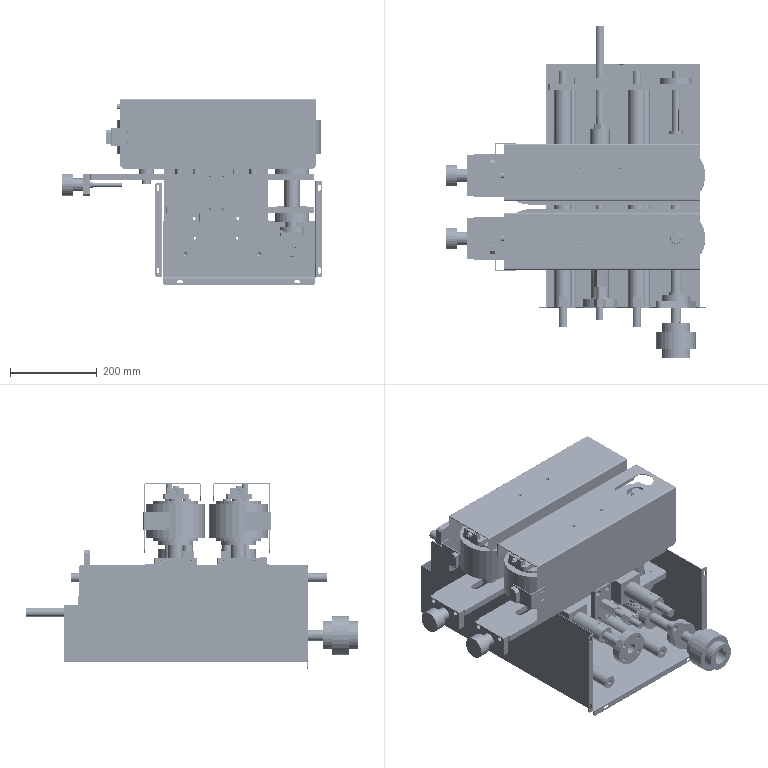Assembly | SolidWorks | mm | 121 component files | 121 solids | 5786 faces | box 600 x 763.5 x 427 mm | volume 18234957 mm3 | cylinder 1615 | torus 1437 | plane 1034 | sphere 814 | spline 504 | cone 382 | commonest cylinder face diameters 11 x120 20 x107 9 x88 17 x76 5 x68 6.8 x66 30 x66 8.5 x64
Bill of materials:
Rolling bearings 6004 GB 276-94 | 13 |  | Annular ring assembly that looks like a radial ball bearing: a thin outer ring and an inner ring, both plain cylinders, sharing an axis, with a single row of spherical balls between them.
'-6004BearingHousing | 1 |  | Flat annular disc with a large central bore and four equally spaced small through holes on a circle between the bore and the outer edge.
ref6 | 8 |  | Ball-bearing-like assembly: concentric outer and inner rings with a single row of about 20 balls between them, and rounded ring edges.
6006BearingHousing | 4 |  | Thick annular ring (spacer- or flange-like shape) with a large central bore and four equally spaced counterbored through holes.
'-BeltTensionBlock | 2 |  | Rectangular block with two counterbored vertical through holes near its ends and one larger horizontal through hole crossing the middle of the long side face.
'-BeltTensionHandwheel | 2 |  | Stepped cylindrical bushing-like part with a larger-diameter section and a coaxial smaller-diameter spigot, with an axial bore visible at the small end.
'-BeltTensionScrewRod | 2 |  | Solid cylindrical pin or shaft with a short, raised, larger-diameter collar near one end. The shaft segments on either side of the collar have slightly different diameters.
'-CoverTopPost | 4 |  | Long slender cylindrical rod with an axial hole at one end and a reduced-diameter stepped spigot at the other end.
'-CylinderConnectionSeat | 1 |  | Block with a T-shaped profile: a wide rectangular top plate with chamfered corners and four vertical through holes, above a narrower lower body that has a horizontal through hole and chamfered lower corners.
deep groove ball bearings gb | 3 |  | Ball-bearing-like assembly: concentric outer and inner rings with a single row of about 14 balls, and rounded ring edges.
'-DrivenPulley | 2 |  | Cylindrical sleeve with a central through bore and a short reduced-outer-diameter step at one end.
'-DrivenPulleyShaft | 2 |  | Multi-stepped shaft with a flatted end tang containing a cross hole, a short collar with a groove-like line, a long main body, a larger-diameter band, and reduced, flatted sections at the opposite end.
'-DrivePulleyStopSleeve | 2 |  | Short, thin-walled cylindrical ring or tube section with plain inner and outer diameters.
'-F-M16150F | 1 |  | Stepped, axially symmetric body: a large chamfered cylinder with a hexagonal prism at one end and a series of smaller coaxial steps leading to a long, slender cylindrical shaft at the other end.
'-GuideBushing | 8 |  | Thin-walled, open-ended cylindrical tube or sleeve of constant diameter.
'-GuidePost | 2 |  | Long, slender cylindrical pin or shaft with reduced-diameter journals at both ends and an extra short shoulder step near one end.
'-LimitScrewRod | 1 |  | Hex-headed rod: a long plain cylindrical shank with a short hexagonal head at one end, in the general form of a hex bolt or screw.
'-LimitScrewSleeve | 1 |  | Flanged tube or spigot: a long cylindrical tube joined to a circular flange with a central bore and four bolt holes.
'-LowerGuard | 1 |  | Bent sheet-metal bracket or cover: a top web with one long side flange and one short side flange (an uneven channel), with small holes and an obround slot.
'-LowerSlideSleeveConnectionPlate01 | 1 |  | Rectangular flat plate with chamfered corners, eight through holes in two 2x2 groups, and a large central hole surrounded by four small holes near one end.
'-LowerSlideSleeveConnectionPlate02 | 1 |  | Long, narrow flat plate with chamfered corners and many features: an elongated slot, several groups of round holes in different sizes, and a large hole with four small holes around it near one end.
'-LowerSlideSleeveConnectionPlate02-1 | 1 |  | Long, narrow flat bar with chamfered corners, an elongated slot and two small holes at one end, two short obround slots and two small round holes along the middle, and a large round hole at the other end.
'-LowerStopBlock | 1 |  | Thick rectangular block or spacer plate with chamfered corners and four through holes near the corners.
M16LocatingScrew | 1 |  | Plain cylindrical rod with a hexagonal collar or nut-like prism at mid-length.
M16Nut | 1 |  | Hexagonal prism with a round through bore along its axis, in the general form of a hex spacer, standoff or coupling sleeve.
'-M30X1.5Nut | 1 |  | Flat, thin annular ring with four rectangular notches cut into the outer edge, spaced evenly around it.
GB_FASTENER_SCREWS_HSHCS M8X60-N | 2 |  | Long, straight cylindrical pin with a short, larger-diameter cylindrical head at one end, like a headed pin or ejector-style pin.
'-MainDrivePulley | 2 |  | Solid cylindrical hub with a central keyed bore and a short, smaller-diameter step at one end.
MaterialDetectionSensor | 2 |  | Rectangular block. Its profile has two rounded corners and one angled corner. Two round holes pass through near one edge.
MaterialDetectionSensorMountingPlate | 2 |  | L-shaped bracket bent from sheet, with a uniform thin wall, an inside bend radius, and two elongated slots in each leg.
'-MovingBushing | 4 |  | Rectangular block with a large round bore running along its long axis and four small holes in a rectangular pattern on one long face.
'-MovingSleeve | 1 |  | Tubular sleeve with a stepped outer diameter, an internal keyway, and a small notch in the outer rim at one end.
ref3 | 3 |  | Straight-tooth bevel gear with a cylindrical hub on its back, a keyed central bore, and small radial holes in the hub.
'-PullerDriveShaft | 1 |  | Long, slender stepped shaft with two main diameters, several keyseats along its length, and chamfered ends.
SC-63X100PistonRod | 1 |  | Stepped cylindrical pin or shaft: a long main body, a short narrow groove or collar near one end, then a smaller-diameter end stub.
'-SlidingBearingHousing | 1 |  | Thick rectangular plate with one large round hole near one end, three small holes in a row at the other end, and two chamfered corners at the large-hole end.
'-SmallPulley | 6 |  | Plain cylindrical tube or sleeve with a uniform outer diameter and a large through-bore.
'-SmallPulleyBearingHousing | 6 |  | Rectangular base plate with two through holes and a centered upright stepped post: a larger-diameter collar, then a long smaller pin with a groove near the tip.
'-SmallSupport | 4 |  | Slender cylindrical rod with a small axial hole in one end face. The other end steps down to a short pin of smaller diameter, and the section next to that pin has a flat cut on one side.
'-SpacerPlate | 1 |  | Rectangular block with three evenly spaced round through-holes in a row across one long side face.
'-TighteningHandwheelBasePlate | 2 |  | Thick rectangular plate with one larger central hole, two smaller holes near the top corners, and chamfered bottom corners.
'-TopPlateSupport | 2 |  | Long thin cylindrical tube or rod with a small concentric hole in the end face.
'-TractionBelt | 2 |  | Thin-walled open loop shaped like a stadium (obround): two straight sides joined by semicircular ends, with a constant wall height and open top and bottom.
ref29 | 1 |  | Straight-tooth bevel gear with a cylindrical hub, a central bore with a keyway, and a small radial hole through the hub.
TractorCoupling | 1 |  | Stepped cylindrical body: a larger-diameter center section with a smaller cylindrical hub on each side, and a central through-bore with a keyway.
'-TractorCover | 1 |  | Sheet-metal tray or enclosure: flat base, two tall side walls with outward mounting flanges that have slotted holes, a lower back wall with a rectangular notch that has rounded corners, and a bottom-edge flange with slots.
'-TractorDriveShaft | 2 |  | Stepped round shaft with several diameter sections: a larger central section, smaller sections stepping down toward one end, and narrow grooves near the other end.
'-TractorTopPlate | 1 |  | Flat L-shaped (stepped) plate with chamfered corners. It has a large central obround slot surrounded by four small holes and four larger corner holes, plus a smaller round hole with four small holes around it on the extended lower portion.
'-UCFL205 | 1 |  | Two-hole diamond-shaped flange with rounded ends, a central through-bore, and a stepped cylindrical boss on one face.
'-UpperGuard | 1 |  | Bent sheet-metal cover with an inverted-U or channel profile: a flat top and two downturned legs of unequal length, with rounded bends.
'-UpperPullCylinderMountingPlate | 1 |  | Rectangular flat plate with small chamfered corners, a large central round through-hole, four round through-holes in a rectangular pattern, and four elongated through-slots (two near each short edge), oriented across the plate's long direction.
'-UpperSlidingSleeveConnectingPlate01 | 1 |  | Elongated rectangular flat plate with small chamfered corners, a large round through-hole near one end surrounded by four small holes in a square pattern, plus several patterns of medium and small through-holes along the rest of the plate.
'-UpperSlidingSleeveConnectingPlate02 | 1 |  | Long narrow flat plate with small chamfered corners. It has one long obround slot near one end, a large round through-hole with four small surrounding holes near the other end, and two roughly mirrored clusters of medium and small round holes in between.
'-UpperSlidingSleeveConnectingPlate02-1 | 1 |  | Long narrow flat bar with chamfered corners. It has a long obround slot near one end with two small holes at that end edge, a central row of two small round holes and two short obround slots, and a large round through-hole near the other end.
Mates:
1. parallel | -GuidePost-3 plane at (-55, 1481, -40) dir (0, 0, 1) | assembly plane at (0, 0, 0) dir (0, 0, 1)
2. parallel | -GuidePost-4 plane at (115, 1481, -40) dir (0, 0, 1) | assembly plane at (0, 0, 0) dir (0, 0, 1)
3. concentric | -GuideBushing-1 face at (-55, 1084.5, -40) dir (0, 1, 0) r 22 | -GuideBushing-2 face at (-55, 1024.5, -40) dir (0, 1, 0) r 22
4. concentric | -MovingBushing-1 face at (-55, 1144.5, -40) dir (0, -1, 0) r 22 | -GuideBushing-2 face at (-55, 1024.5, -40) dir (0, 1, 0) r 22
5. coincident | -MovingBushing-1 face at (-55, 1024.5, -40) dir (0, -1, 0) | -GuideBushing-2 face at (-55, 1024.5, -40) dir (0, -1, 0)
6. coincident | -MovingBushing-1 face at (-55, 1144.5, -40) dir (0, 1, 0) | -GuideBushing-1 face at (-55, 1144.5, -40) dir (0, 1, 0)
7. concentric | -GuidePost-3 face at (-55, 4097.332, -40) dir (0, 1, 0) r 20 | -GuideBushing-1 face at (-55, 1084.5, -40) dir (0, 1, 0) r 20
8. concentric | -GuideBushing-3 face at (115, 1084.5, -40) dir (0, 1, 0) r 22 | -GuideBushing-4 face at (115, 1024.5, -40) dir (0, 1, 0) r 22
9. concentric | -MovingBushing-2 face at (115, 1144.5, -40) dir (0, -1, 0) r 22 | -GuideBushing-3 face at (115, 1084.5, -40) dir (0, 1, 0) r 22
10. coincident | -MovingBushing-2 face at (115, 1144.5, -40) dir (0, 1, 0) | -GuideBushing-3 face at (115, 1144.5, -40) dir (0, 1, 0)
11. coincident | -MovingBushing-2 face at (115, 1024.5, -40) dir (0, -1, 0) | -GuideBushing-4 face at (115, 1024.5, -40) dir (0, -1, 0)
12. concentric | -GuidePost-4 face at (115, 4097.332, -40) dir (0, 1, 0) r 20 | -GuideBushing-3 face at (115, 1084.5, -40) dir (0, 1, 0) r 20
13. coincident | -MovingBushing-1 face at (-25, 1144.5, -10) dir (0, 0, 1) | -LowerSlideSleeveConnectionPlate02-1 face at (17.5, 1094.5, -10) dir (0, 0, -1)
14. coincident | -MovingBushing-2 face at (145, 1144.5, -10) dir (0, 0, 1) | -LowerSlideSleeveConnectionPlate02-1 face at (17.5, 1094.5, -10) dir (0, 0, -1)
15. concentric | -MovingBushing-1 face at (-35, 1134.5, -10) dir (0, 0, 1) r 4.25 | -LowerSlideSleeveConnectionPlate02-1 face at (-35, 1134.5, 5) dir (0, 0, 1) r 8.5
16. concentric | -MovingBushing-1 face at (-75, 1134.5, -10) dir (0, 0, 1) r 4.25 | -LowerSlideSleeveConnectionPlate02-1 face at (-75, 1134.5, 5) dir (0, 0, 1) r 8.5
17. concentric | -MovingBushing-2 face at (95, 1134.5, -10) dir (0, 0, 1) r 4.25 | -LowerSlideSleeveConnectionPlate02-1 face at (95, 1134.5, 5) dir (0, 0, 1) r 8.5
18. concentric | -MovingBushing-2 face at (135, 1134.5, -10) dir (0, 0, 1) r 4.25 | -LowerSlideSleeveConnectionPlate02-1 face at (135, 1134.5, 5) dir (0, 0, 1) r 8.5
19. coincident | -LowerSlideSleeveConnectionPlate02-1 face at (17.5, 1094.5, 5) dir (0, 0, 1) | -SmallSupport-1 face at (-55, 1079.5, 5) dir (0, 0, -1)
20. coincident | -SmallSupport-1 face at (-55, 1079.5, 140) dir (0, 0, 1) | -SmallSupport-2 face at (115, 1079.5, 140) dir (0, 0, 1)
21. coincident | -SmallSupport-1 face at (-55, 1079.5, 140) dir (0, 0, 1) | -LowerSlideSleeveConnectionPlate02-1-1 face at (25, 1094.5, 140) dir (0, 0, -1)
22. concentric | -SmallSupport-1 face at (-55, 1079.5, 5) dir (0, 0, 1) r 10 | -LowerSlideSleeveConnectionPlate02-1-1 face at (-55, 1079.5, 144) dir (0, 0, 1) r 7
23. coincident | -LowerSlideSleeveConnectionPlate02-1 face at (17.5, 1094.5, 5) dir (0, 0, 1) | -CoverTopPost-1 face at (-15, 1079.5, 5) dir (0, 0, -1)
24. concentric | -LowerSlideSleeveConnectionPlate02-1 face at (-15, 1079.5, -10) dir (0, 0, -1) r 5 | -CoverTopPost-1 face at (-15, 1079.5, 175) dir (0, 0, -1) r 7.5
25. coincident | -CoverTopPost-1 face at (-15, 1079.5, 175) dir (0, 0, 1) | -CoverTopPost-2 face at (75, 1079.5, 175) dir (0, 0, 1)
26. coincident | -LowerSlideSleeveConnectionPlate02-1 face at (17.5, 1094.5, 5) dir (0, 0, 1) | -SmallRollerAssembly-1/-SmallPulleyBearingHousing-1 face at (-45, 1121, 5) dir (0, 0, -1)
27. concentric | -LowerSlideSleeveConnectionPlate02-1 face at (-70, 1121, 5) dir (0, 0, 1) r 3.4 | -SmallRollerAssembly-1/-SmallPulleyBearingHousing-1 face at (-70, 1121, 20) dir (0, 0, 1) r 7.5
28. concentric | -LowerSlideSleeveConnectionPlate02-1 face at (-20, 1121, 5) dir (0, 0, 1) r 3.4 | -SmallRollerAssembly-1/-SmallPulleyBearingHousing-1 face at (-20, 1121, 20) dir (0, 0, 1) r 4.5
29. concentric | 6006BearingHousing-1 face at (205, 1094.5, 540.921) dir (0, 0, 1) r 27.5 | -6006-1 face at (205, 1094.5, 2.789) dir (0, 0, -1) r 27.5
30. coincident | 6006BearingHousing-1 face at (221.74, 1111.698, 18) dir (0, 0, -1) | -6006-1 face at (205, 1122, 18) dir (0, 0, 1)
31. coincident | -LowerSlideSleeveConnectionPlate02-1 face at (17.5, 1094.5, 5) dir (0, 0, 1) | 6006BearingHousing-1 face at (224.181, 1114.206, 5) dir (0, 0, -1)
32. concentric | -LowerSlideSleeveConnectionPlate02-1 face at (205, 1094.5, -10) dir (0, 0, 1) r 21 | 6006BearingHousing-1 face at (205, 1094.5, 540.921) dir (0, 0, 1) r 40
33. concentric | -LowerSlideSleeveConnectionPlate02-1 face at (228.54, 1118.685, 5) dir (0, 0, 1) r 2.5 | 6006BearingHousing-1 face at (228.54, 1118.685, 25) dir (0, 0, 1) r 3.5
34. concentric | -TractorDriveShaft-1 face at (205, 1094.5, 589.237) dir (0, 0, 1) r 15 | -MainDrivePulley-1 face at (205, 1094.5, 829.122) dir (0, 0, 1) r 15
35. concentric | -TractorDriveShaft-1 face at (205, 1094.5, 589.237) dir (0, 0, 1) r 17.5 | -6006-1 face at (205, 1094.5, 4.529) dir (0, 0, -1) r 15
36. coincident | -TractorDriveShaft-1 face at (193.599, 1104.247, 5) dir (0, 0, 1) | -6006-1 face at (205, 1113.667, 5) dir (0, 0, -1)
37. concentric | -LowerSlideSleeveConnectionPlate02-1-1 face at (205, 1094.5, 152) dir (0, 0, -1) r 23.5 | deep groove ball bearings gb-2 face at (205, 1094.5, 156.711) dir (0, 0, 1) r 13
38. coincident | -LowerSlideSleeveConnectionPlate02-1-1 face at (25, 1094.5, 152) dir (0, 0, 1) | deep groove ball bearings gb-2 face at (205, 1107.5, 152) dir (0, 0, 1)
39. coincident | -TractorDriveShaft-1 face at (193.599, 1104.247, 135) dir (0, 0, 1) | -MainDrivePulley-1 face at (191.144, 1088.754, 135) dir (0, 0, 1)
40. coincident | -6006-1 face at (205, 1109.5, 18) dir (0, 0, 1) | -DrivePulleyStopSleeve-1 face at (205, 1094.5, 18) dir (0, 0, -1)
41. concentric | -TractorDriveShaft-1 face at (205, 1094.5, 589.237) dir (0, 0, 1) r 15 | -DrivePulleyStopSleeve-1 face at (205, 1094.5, 18) dir (0, 0, 1) r 15
42. concentric | -DrivenPulley-1 face at (-130, 1094.5, 829.122) dir (0, 0, 1) r 27.5 | -6006-2 face at (-130, 1094.5, 137.211) dir (0, 0, 1) r 27.5
43. coincident | -DrivenPulley-1 face at (-156.941, 1100.019, 135) dir (0, 0, 1) | -6006-2 face at (-137.283, 1112.229, 135) dir (0, 0, 1)
44. concentric | -DrivenPulley-1 face at (-130, 1094.5, 829.122) dir (0, 0, 1) r 40 | -6006-3 face at (-130, 1094.5, 50.211) dir (0, 0, 1) r 27.5
45. coincident | -DrivenPulley-1 face at (-169.186, 1102.527, 35) dir (0, 0, -1) | -6006-3 face at (-140.449, 1119.937, 35) dir (0, 0, -1)
46. concentric | -DrivenPulleyShaft-1 face at (-130, 1094.5, 681.379) dir (0, 0, 1) r 15 | -DrivenPulley-1 face at (-130, 1094.5, 829.122) dir (0, 0, 1) r 52.5
47. coincident | -LowerSlideSleeveConnectionPlate02-1 face at (-175, 1084.5, -10) dir (0, 1, 0) | -DrivenPulleyShaft-1 face at (-144.635, 1084.5, 5) dir (0, -1, 0)
48. coincident | -LowerSlideSleeveConnectionPlate02-1 face at (17.5, 1094.5, 5) dir (0, 0, 1) | -DrivenPulleyShaft-1 face at (-130, 1077, 5) dir (0, 0, -1)
49. coincident | -LowerSlideSleeveConnectionPlate02-1 plane at (-130, 1094.5, -2.5) dir (-1, 0, 0) | -DrivenPulleyShaft-1 plane at (-130, 1094.5, 170) dir (-1, 0, 0)
50. coincident | -LowerSlideSleeveConnectionPlate02-1 face at (-260, 1144.5, 5) dir (-1, 0, 0) | -TighteningHandwheelBasePlate-1 face at (-260, 1094.5, -20) dir (1, 0, 0)
51. concentric | -LowerSlideSleeveConnectionPlate02-1 face at (-260, 1129.5, -2.5) dir (-1, 0, 0) r 2.5 | -TighteningHandwheelBasePlate-1 face at (-275, 1129.5, -2.5) dir (-1, 0, 0) r 5.5
52. concentric | -LowerSlideSleeveConnectionPlate02-1 face at (-260, 1059.5, -2.5) dir (-1, 0, 0) r 2.5 | -TighteningHandwheelBasePlate-1 face at (-275, 1059.5, -2.5) dir (-1, 0, 0) r 5.5
53. concentric | -TighteningHandwheelBasePlate-1 face at (-260, 1094.5, -20) dir (-1, 0, 0) r 6 | -BeltTensionScrewRod-1 face at (-749.959, 1094.5, -20) dir (-1, 0, 0) r 6
54. coincident | -MovingBushing-1 face at (-25, 1144.5, -70) dir (0, 0, -1) | -LowerSlideSleeveConnectionPlate01-1 face at (85, 1094.5, -70) dir (0, 0, 1)
55. concentric | -MovingBushing-2 face at (95, 1134.5, -70) dir (0, 0, -1) r 4.25 | -LowerSlideSleeveConnectionPlate01-1 face at (95, 1134.5, -85) dir (0, 0, -1) r 8.5
56. concentric | -MovingBushing-2 face at (135, 1134.5, -70) dir (0, 0, -1) r 4.25 | -LowerSlideSleeveConnectionPlate01-1 face at (135, 1134.5, -85) dir (0, 0, -1) r 8.5
57. coincident | -LowerSlideSleeveConnectionPlate02-1-1 face at (25, 1094.5, 152) dir (0, 0, 1) | -BeltTensionBlock-1 face at (-190, 1114.5, 152) dir (0, 0, -1)
58. concentric | -LowerSlideSleeveConnectionPlate02-1-1 face at (-184, 1107.5, 152) dir (0, 0, 1) r 2.5 | -BeltTensionBlock-1 face at (-184, 1107.5, 167) dir (0, 0, 1) r 5.5
59. concentric | -LowerSlideSleeveConnectionPlate02-1-1 face at (-184, 1081.5, 152) dir (0, 0, 1) r 2.5 | -BeltTensionBlock-1 face at (-184, 1081.5, 167) dir (0, 0, 1) r 3.5
60. concentric | -GuideBushing-5 face at (-55, 1189.5, -40) dir (0, 1, 0) r 22 | -GuideBushing-6 face at (-55, 1249.5, -40) dir (0, 1, 0) r 22
61. coincident | -MovingBushing-3 face at (-55, 1189.5, -40) dir (0, -1, 0) | -GuideBushing-5 face at (-55, 1189.5, -40) dir (0, -1, 0)
62. coincident | -MovingBushing-3 face at (-55, 1309.5, -40) dir (0, 1, 0) | -GuideBushing-6 face at (-55, 1309.5, -40) dir (0, 1, 0)
63. concentric | -MovingBushing-3 face at (-55, 1189.5, -40) dir (0, 1, 0) r 22 | -GuideBushing-6 face at (-55, 1249.5, -40) dir (0, 1, 0) r 22
64. concentric | -GuidePost-3 face at (-55, 4097.332, -40) dir (0, 1, 0) r 20 | -GuideBushing-6 face at (-55, 1249.5, -40) dir (0, 1, 0) r 20
65. concentric | -MovingBushing-4 face at (115, 1189.5, -40) dir (0, 1, 0) r 22 | -GuideBushing-8 face at (115, 1249.5, -40) dir (0, -1, 0) r 22
66. coincident | -MovingBushing-4 face at (115, 1189.5, -40) dir (0, -1, 0) | -GuideBushing-8 face at (115, 1189.5, -40) dir (0, -1, 0)
67. concentric | -GuideBushing-7 face at (115, 1249.5, -40) dir (0, 1, 0) r 22 | -GuideBushing-8 face at (115, 1249.5, -40) dir (0, -1, 0) r 20
68. coincident | -MovingBushing-4 face at (115, 1309.5, -40) dir (0, 1, 0) | -GuideBushing-7 face at (115, 1309.5, -40) dir (0, 1, 0)
69. concentric | -GuidePost-4 face at (115, 4097.332, -40) dir (0, 1, 0) r 20 | -GuideBushing-8 face at (115, 1249.5, -40) dir (0, -1, 0) r 20
70. coincident | -MovingBushing-3 face at (-25, 1189.5, -10) dir (0, 0, 1) | -UpperSlidingSleeveConnectingPlate02-1 face at (-2.5, 1239.5, -10) dir (0, 0, -1)
71. concentric | -MovingBushing-4 face at (135, 1274.5, -10) dir (0, 0, 1) r 4.25 | -UpperSlidingSleeveConnectingPlate02-1 face at (135, 1274.5, 5) dir (0, 0, 1) r 8.5
72. coincident | -MovingBushing-4 face at (85, 1189.5, -10) dir (0, 0, 1) | -UpperSlidingSleeveConnectingPlate02-1 face at (-2.5, 1239.5, -10) dir (0, 0, -1)
73. concentric | -MovingBushing-3 face at (-35, 1274.5, -10) dir (0, 0, 1) r 4.25 | -UpperSlidingSleeveConnectingPlate02-1 face at (-35, 1274.5, 5) dir (0, 0, 1) r 8.5
74. concentric | -MovingBushing-3 face at (-75, 1274.5, -10) dir (0, 0, 1) r 4.25 | -UpperSlidingSleeveConnectingPlate02-1 face at (-75, 1274.5, 5) dir (0, 0, 1) r 8.5
75. coincident | -UpperSlidingSleeveConnectingPlate02-1 face at (-2.5, 1239.5, 5) dir (0, 0, 1) | -SmallSupport-3 face at (-55, 1254.5, 5) dir (0, 0, -1)
76. coincident | -UpperSlidingSleeveConnectingPlate02-1 face at (-2.5, 1239.5, 5) dir (0, 0, 1) | -CoverTopPost-4 face at (-15, 1254.5, 5) dir (0, 0, -1)
77. coincident | -UpperSlidingSleeveConnectingPlate02-1 face at (-2.5, 1239.5, 5) dir (0, 0, 1) | -CoverTopPost-5 face at (75, 1254.5, 5) dir (0, 0, -1)
78. coincident | -UpperSlidingSleeveConnectingPlate02-1 face at (-2.5, 1239.5, 5) dir (0, 0, 1) | -SmallSupport-4 face at (115, 1254.5, 5) dir (0, 0, -1)
79. coincident | -SmallSupport-3 face at (-55, 1254.5, 140) dir (0, 0, 1) | -UpperSlidingSleeveConnectingPlate02-1-1 face at (25, 1239.5, 140) dir (0, 0, -1)
80. concentric | -SmallSupport-3 face at (-55, 1254.5, 5) dir (0, 0, 1) r 10 | -UpperSlidingSleeveConnectingPlate02-1-1 face at (-55, 1254.5, 144) dir (0, 0, 1) r 7
81. coincident | -UpperSlidingSleeveConnectingPlate02-1 face at (-2.5, 1239.5, 5) dir (0, 0, 1) | -SmallRollerAssembly-4/-SmallPulleyBearingHousing-1 face at (-45, 1213, 5) dir (0, 0, -1)
82. concentric | -UpperSlidingSleeveConnectingPlate02-1 face at (-20, 1213, 5) dir (0, 0, 1) r 3.4 | -SmallRollerAssembly-4/-SmallPulleyBearingHousing-1 face at (-20, 1213, 20) dir (0, 0, 1) r 7.5
83. concentric | -UpperSlidingSleeveConnectingPlate02-1 face at (-70, 1213, 5) dir (0, 0, 1) r 3.4 | -SmallRollerAssembly-4/-SmallPulleyBearingHousing-1 face at (-70, 1213, 20) dir (0, 0, 1) r 4.5
84. coincident | 6006BearingHousing-2 face at (221.971, 1256.471, 18) dir (0, 0, -1) | -6006-4 face at (205, 1267, 18) dir (0, 0, 1)
85. concentric | 6006BearingHousing-2 face at (205, 1239.5, 540.921) dir (0, 0, 1) r 24 | -6006-4 face at (205, 1239.5, 2.789) dir (0, 0, -1) r 27.5
86. coincident | -UpperSlidingSleeveConnectingPlate02-1 face at (-2.5, 1239.5, 5) dir (0, 0, 1) | 6006BearingHousing-2 face at (224.445, 1258.945, 5) dir (0, 0, -1)
87. concentric | -UpperSlidingSleeveConnectingPlate02-1 face at (181.135, 1263.365, 5) dir (0, 0, 1) r 2.5 | 6006BearingHousing-2 face at (181.135, 1263.365, 25) dir (0, 0, 1) r 5.5
88. concentric | -UpperSlidingSleeveConnectingPlate02-1 face at (228.865, 1263.365, 5) dir (0, 0, 1) r 2.5 | 6006BearingHousing-2 face at (228.865, 1263.365, 25) dir (0, 0, 1) r 5.5
89. concentric | -MainDrivePulley-2 face at (205, 1239.5, 829.122) dir (0, 0, 1) r 52.5 | -TractorDriveShaft-2 face at (205, 1239.5, 589.237) dir (0, 0, 1) r 15
90. concentric | -TractorDriveShaft-2 face at (205, 1239.5, 589.237) dir (0, 0, 1) r 15 | -DrivePulleyStopSleeve-2 face at (205, 1239.5, 18) dir (0, 0, 1) r 17.5
91. coincident | -MainDrivePulley-2 face at (210.53, 1199.884, 35) dir (0, 0, -1) | -DrivePulleyStopSleeve-2 face at (205, 1239.5, 35) dir (0, 0, 1)
92. coincident | -6006-4 face at (205, 1254.5, 18) dir (0, 0, 1) | -DrivePulleyStopSleeve-2 face at (205, 1239.5, 18) dir (0, 0, -1)
93. concentric | -6006-4 face at (205, 1239.5, 4.529) dir (0, 0, -1) r 15 | -TractorDriveShaft-2 face at (205, 1239.5, 589.237) dir (0, 0, 1) r 17.5
94. coincident | -6006-4 face at (205, 1258.667, 5) dir (0, 0, -1) | -TractorDriveShaft-2 face at (202.563, 1254.301, 5) dir (0, 0, 1)
95. concentric | -TractorDriveShaft-2 face at (205, 1239.5, 589.237) dir (0, 0, 1) r 12.5 | deep groove ball bearings gb-4 face at (205, 1239.5, 141.029) dir (0, 0, -1) r 5
96. coincident | -UpperSlidingSleeveConnectingPlate02-1-1 face at (25, 1239.5, 152) dir (0, 0, 1) | deep groove ball bearings gb-4 face at (205, 1252.5, 152) dir (0, 0, 1)
97. concentric | -MovingBushing-4 face at (135, 1274.5, -70) dir (0, 0, -1) r 4.25 | -UpperSlidingSleeveConnectingPlate01-1 face at (135, 1274.5, -85) dir (0, 0, -1) r 8.5
98. concentric | -MovingBushing-4 face at (95, 1274.5, -70) dir (0, 0, -1) r 4.25 | -UpperSlidingSleeveConnectingPlate01-1 face at (95, 1274.5, -85) dir (0, 0, -1) r 8.5
99. coincident | -MovingBushing-4 face at (85, 1189.5, -70) dir (0, 0, -1) | -UpperSlidingSleeveConnectingPlate01-1 face at (85, 1239.5, -70) dir (0, 0, 1)
100. coincident | -DrivenPulley-2 face at (-130, 1239.5, 829.122) dir (0, 0, 1) r 27.5 | -6006-5 edge at (-130, 1239.5, 123) dir (0, 0, 1) r 27.5
101. coincident | -DrivenPulley-2 face at (-116.217, 1215.704, 135) dir (0, 0, 1) | -6006-5 face at (-137.283, 1257.229, 135) dir (0, 0, 1)
102. concentric | -DrivenPulley-2 face at (-130, 1239.5, 829.122) dir (0, 0, 1) r 27.5 | -6006-6 face at (-130, 1239.5, 50.211) dir (0, 0, 1) r 27.5
103. coincident | -DrivenPulley-2 face at (-109.951, 1204.887, 35) dir (0, 0, -1) | -6006-6 face at (-140.449, 1264.937, 35) dir (0, 0, -1)
104. concentric | -6006-5 face at (-130, 1239.5, 135.471) dir (0, 0, 1) r 15 | -DrivenPulleyShaft-2 face at (-130, 1239.5, 681.379) dir (0, 0, 1) r 15
105. coincident | -6006-5 face at (-137.283, 1257.229, 135) dir (0, 0, 1) | -DrivenPulleyShaft-2 face at (-130, 1226, 135) dir (0, 0, 1)
106. coincident | -UpperSlidingSleeveConnectingPlate02-1 face at (-175, 1249.5, -10) dir (0, -1, 0) | -DrivenPulleyShaft-2 face at (-144.635, 1249.5, 5) dir (0, 1, 0)
107. coincident | -UpperSlidingSleeveConnectingPlate02-1 face at (-2.5, 1239.5, 5) dir (0, 0, 1) | -DrivenPulleyShaft-2 face at (-130, 1222, 5) dir (0, 0, -1)
108. coincident | -DrivenPulleyShaft-1 plane at (-130, 1094.5, 170) dir (-1, 0, 0) | -DrivenPulleyShaft-2 plane at (-130, 1239.5, 170) dir (-1, 0, 0)
109. coincident | -UpperSlidingSleeveConnectingPlate02-1-1 face at (25, 1239.5, 152) dir (0, 0, 1) | -BeltTensionBlock-2 face at (-190, 1259.5, 152) dir (0, 0, -1)
110. concentric | -UpperSlidingSleeveConnectingPlate02-1-1 face at (-184, 1252.5, 152) dir (0, 0, 1) r 2.5 | -BeltTensionBlock-2 face at (-184, 1252.5, 167) dir (0, 0, 1) r 5.5
111. concentric | -UpperSlidingSleeveConnectingPlate02-1-1 face at (-184, 1226.5, 152) dir (0, 0, 1) r 2.5 | -BeltTensionBlock-2 face at (-184, 1226.5, 167) dir (0, 0, 1) r 3.5
112. coincident | -UpperSlidingSleeveConnectingPlate02-1 face at (-260, 1189.5, 5) dir (-1, 0, 0) | -TighteningHandwheelBasePlate-2 face at (-260, 1239.5, -20) dir (1, 0, 0)
113. concentric | -UpperSlidingSleeveConnectingPlate02-1 face at (-260, 1274.5, -2.5) dir (-1, 0, 0) r 2.5 | -TighteningHandwheelBasePlate-2 face at (-275, 1274.5, -2.5) dir (-1, 0, 0) r 5.5
114. concentric | -UpperSlidingSleeveConnectingPlate02-1 face at (-260, 1204.5, -2.5) dir (-1, 0, 0) r 2.5 | -TighteningHandwheelBasePlate-2 face at (-275, 1204.5, -2.5) dir (-1, 0, 0) r 3.5
115. concentric | -GuidePost-3 face at (-55, 4097.332, -40) dir (0, 1, 0) r 10 | -TractorTopPlate-1 face at (-55, 1436, -40) dir (0, 1, 0) r 10.5
116. coincident | -GuidePost-3 face at (-55, 1436, -50) dir (0, 1, 0) | -TractorTopPlate-1 face at (150, 1436, 22.5) dir (0, -1, 0)
117. concentric | -GuidePost-4 face at (115, 4097.332, -40) dir (0, 1, 0) r 10 | -TractorTopPlate-1 face at (115, 1436, -40) dir (0, 1, 0) r 10.5
118. concentric | -TractorTopPlate-1 face at (130, 1436, -180) dir (0, 1, 0) r 6.5 | -TopPlateSupport-1 face at (130, 1436, -180) dir (0, -1, 0) r 15
119. coincident | -TractorTopPlate-1 face at (150, 1436, 22.5) dir (0, -1, 0) | -TopPlateSupport-1 face at (130, 1436, -180) dir (0, 1, 0)
120. coincident | -TractorTopPlate-1 face at (150, 1436, 22.5) dir (0, -1, 0) | -TopPlateSupport-2 face at (-40, 1436, -180) dir (0, 1, 0)
121. concentric | -TractorTopPlate-1 face at (-40, 1436, -180) dir (0, 1, 0) r 6.5 | -TopPlateSupport-2 face at (-40, 1436, -180) dir (0, -1, 0) r 15
122. concentric | -UpperSlidingSleeveConnectingPlate01-1 face at (180, 1289.5, -77.5) dir (0, 1, 0) r 3.4 | -SpacerPlate-1 face at (180, 1309.5, -77.5) dir (0, 1, 0) r 4.5
123. concentric | -UpperSlidingSleeveConnectingPlate01-1 face at (205, 1289.5, -77.5) dir (0, 1, 0) r 3.4 | -SpacerPlate-1 face at (205, 1309.5, -77.5) dir (0, 1, 0) r 4.5
124. coincident | -UpperSlidingSleeveConnectingPlate01-1 face at (-85, 1289.5, -70) dir (0, 1, 0) | -SpacerPlate-1 face at (240, 1289.5, -70) dir (0, -1, 0)
125. concentric | -SpacerPlate-1 face at (230, 1309.5, -77.5) dir (0, 1, 0) r 4.5 | -SlidingBearingHousing-1 face at (230, 1309.5, -77.5) dir (0, 1, 0) r 4.5
126. coincident | -SpacerPlate-1 face at (240, 1309.5, -70) dir (0, 1, 0) | -SlidingBearingHousing-1 face at (205, 1309.5, -139) dir (0, -1, 0)
127. concentric | -SpacerPlate-1 face at (205, 1309.5, -77.5) dir (0, 1, 0) r 4.5 | -SlidingBearingHousing-1 face at (205, 1309.5, -77.5) dir (0, 1, 0) r 4.5
128. coincident | -SlidingBearingHousing-1 face at (205, 1313.5, -198) dir (0, 1, 0) | deep groove ball bearings gb-5 face at (217.527, 1313.5, -169.525) dir (0, -1, 0)
129. concentric | -SlidingBearingHousing-1 face at (205, 1277.242, -173) dir (0, -1, 0) r 29 | deep groove ball bearings gb-5 face at (205, 1326.211, -173) dir (0, 1, 0) r 13
130. concentric | -PullerDriveShaft-1 face at (205, -3142.913, -173) dir (0, -1, 0) r 10 | -MovingSleeve-1 face at (205, -2057.705, -173) dir (0, -1, 0) r 10
131. coincident | deep groove ball bearings gb-5 face at (212.388, 1321.5, -170.951) dir (0, 1, 0) | -M30X1.5Nut-1 face at (205, 1321.5, -173) dir (0, -1, 0)
132. concentric | -MovingSleeve-1 face at (205, -2057.705, -173) dir (0, -1, 0) r 15 | -M30X1.5Nut-1 face at (205, 1321.5, -173) dir (0, 1, 0) r 20
133. concentric | -TractorDriveShaft-2 face at (205, 1239.5, 589.237) dir (0, 0, 1) r 12.5 | -6006-7 face at (205, 1239.5, -84.529) dir (0, 0, 1) r 15
134. concentric | -UpperSlidingSleeveConnectingPlate01-1 face at (181.135, 1263.365, -70) dir (0, 0, 1) r 2.5 | 6006BearingHousing-3 face at (181.135, 1263.365, -105) dir (0, 0, -1) r 5.5
135. concentric | -UpperSlidingSleeveConnectingPlate01-1 face at (228.865, 1263.365, -70) dir (0, 0, 1) r 2.5 | 6006BearingHousing-3 face at (228.865, 1263.365, -105) dir (0, 0, -1) r 5.5
136. coincident | -6006-7 face at (205, 1267, -98) dir (0, 0, -1) | 6006BearingHousing-3 face at (188.029, 1256.471, -98) dir (0, 0, 1)
137. coincident | -TractorDriveShaft-2 face at (202.563, 1254.301, -85) dir (0, 0, -1) | -6006-7 face at (205, 1258.667, -85) dir (0, 0, 1)
138. coincident | 6006BearingHousing-4 face at (188.029, 1077.529, -98) dir (0, 0, 1) | -6006-8 face at (205, 1067, -98) dir (0, 0, -1)
139. concentric | 6006BearingHousing-4 face at (205, 1094.5, -620.921) dir (0, 0, -1) r 40 | -6006-8 face at (205, 1094.5, -82.789) dir (0, 0, 1) r 27.5
140. coincident | -LowerSlideSleeveConnectionPlate01-1 face at (85, 1094.5, -85) dir (0, 0, -1) | 6006BearingHousing-4 face at (185.555, 1075.055, -85) dir (0, 0, 1)
141. concentric | -LowerSlideSleeveConnectionPlate01-1 face at (181.135, 1118.365, -70) dir (0, 0, 1) r 2.5 | 6006BearingHousing-4 face at (181.135, 1118.365, -105) dir (0, 0, -1) r 5.5
142. concentric | -LowerSlideSleeveConnectionPlate01-1 face at (228.865, 1118.365, -70) dir (0, 0, 1) r 2.5 | 6006BearingHousing-4 face at (228.865, 1118.365, -105) dir (0, 0, -1) r 5.5
143. coincident | -UpperGuard-1 face at (260, 1186.5, 175) dir (0, 0, -1) | -CoverTopPost-4 face at (-15, 1254.5, 175) dir (0, 0, 1)
144. coincident | -TractorTopPlate-1 face at (150, 1451, 22.5) dir (0, 1, 0) | -6004BearingHousing-1 face at (242, 1451, -173) dir (0, -1, 0)
145. concentric | -TractorTopPlate-1 edge at (205, 1451, -143) dir (0, 1, 0) r 2.5 | -6004BearingHousing-1 face at (205, 1465, -143) dir (0, -1, 0) r 3.5
146. distance | -6004-1 face at (226, 1453, -173) dir (0, -1, 0) | -TractorTopPlate-1 face at (150, 1451, 22.5) dir (0, 1, 0)
147. concentric | -BeltTensionScrewRod-1 face at (-749.959, 1094.5, -20) dir (-1, 0, 0) r 6 | -BeltTensionHandwheel-1 face at (-794.095, 1094.5, -20) dir (-1, 0, 0) r 25
148. coincident | -BeltTensionScrewRod-1 face at (-290, 1107.091, -33.5) dir (-1, 0, 0) | -BeltTensionHandwheel-1 face at (-290, 1088.551, -20.782) dir (1, 0, 0)
149. concentric | -TractorDriveShaft-2 face at (205, 1239.5, 589.237) dir (0, 0, 1) r 12.5 | -PullerBevelGear02-1 face at (205, 1239.5, -194.124) dir (0, 0, 1) r 12.5
150. coincident | -TractorDriveShaft-2 face at (212.737, 1244.828, -123) dir (0.1624, -0.9867, 0) | -PullerBevelGear02-1 face at (219.94, 1246.014, -194.124) dir (0.1624, -0.9867, 0)
151. coincident | -PullerBevelGear02-1 sketch point at (205, 1239.5, -173) dir (1, 0, 0) | -TractorBevelGear01-1 sketch point at (205, 1239.5, -173) dir (1, 0, 0)
152. coincident | -MovingSleeve-1 face at (201.084, 1261.878, -182.202) dir (0, -1, 0) | -TractorBevelGear01-1 face at (205, 1261.878, -173) dir (0, -1, 0)
153. coincident | -PullerDriveShaft-1 face at (210.306, 1390, -168.194) dir (-0.9202, 0, 0.3916) | -MovingSleeve-1 face at (212.851, 1341.878, -162.213) dir (-0.9202, 0, 0.3916)
154. perpendicular | -PullerBevelGear02-1 sketch segment at (205, 1239.5, -129.124) dir (0, 0, -1) | -TractorBevelGear01-1 sketch segment at (205, 1283.376, -173) dir (0, -1, 0)
155. concentric | -PullerDriveShaft-1 face at (205, -3142.913, -173) dir (0, -1, 0) r 10 | -TractorBevelGear01-1 face at (205, 1294.5, -173) dir (0, -1, 0) r 28
156. distance | -PullerBevelGear02-1 face at (205, 1239.5, -150.622) dir (0, 0, -1) | -TractorDriveShaft-2 face at (202.969, 1251.834, -153) dir (0, 0, -1)
157. concentric | -TractorDriveShaft-1 face at (205, 1094.5, 589.237) dir (0, 0, 1) r 12.5 | -PullerBevelGear02-2 face at (205, 1094.5, -118) dir (0, 0, -1) r 28
158. concentric | -PullerDriveShaft-1 face at (205, 1479.7, -173) dir (0, 1, 0) r 12.5 | -PullerBevelGear02-3 face at (205, 1039.5, -173) dir (0, 1, 0) r 28
159. coincident | -PullerBevelGear02-2 sketch point at (205, 1094.5, -173) dir (1, 0, 0) | -PullerBevelGear02-3 sketch point at (205, 1094.5, -173) dir (1, 0, 0)
160. coincident | -PullerBevelGear02-1 face at (205, 1239.5, -150.622) dir (0, 0, -1) | -PullerBevelGear02-2 face at (205, 1094.5, -150.622) dir (0, 0, -1)
161. concentric | -CoverTopPost-2 face at (75, 1079.5, 175) dir (0, 0, -1) r 7.5 | -LowerGuard-1 face at (75, 1079.5, 167) dir (0, 0, 1) r 4
162. coincident | -CoverTopPost-2 face at (75, 1079.5, 175) dir (0, 0, 1) | -LowerGuard-1 face at (-190, 1147.5, 175) dir (0, 0, -1)
163. concentric | -UpperSlidingSleeveConnectingPlate02-1-1 face at (205, 1239.5, 152) dir (0, 0, -1) r 23.5 | deep groove ball bearings gb-4 face at (205, 1239.5, 139.289) dir (0, 0, -1) r 13
164. concentric | -SmallSupport-2 face at (115, 1079.5, 140) dir (0, 0, 1) r 3.4 | -LowerSlideSleeveConnectionPlate02-1-1 face at (115, 1079.5, 144) dir (0, 0, 1) r 7
165. concentric | -UpperSlidingSleeveConnectingPlate02-1 face at (-15, 1254.5, -10) dir (0, 0, -1) r 5 | -CoverTopPost-4 face at (-15, 1254.5, 175) dir (0, 0, -1) r 7.5
166. concentric | -UpperSlidingSleeveConnectingPlate02-1 face at (-55, 1254.5, -10) dir (0, 0, -1) r 5 | -SmallSupport-3 face at (-55, 1254.5, 5) dir (0, 0, 1) r 10
167. concentric | -UpperSlidingSleeveConnectingPlate02-1 face at (75, 1254.5, -10) dir (0, 0, -1) r 5 | -CoverTopPost-5 face at (75, 1254.5, 175) dir (0, 0, -1) r 7.5
168. concentric | -CoverTopPost-1 face at (-15, 1079.5, 175) dir (0, 0, 1) r 2.5 | -LowerGuard-1 face at (-15, 1079.5, 167) dir (0, 0, 1) r 4
169. concentric | -UpperGuard-1 face at (-15, 1254.5, 167) dir (0, 0, 1) r 4 | -CoverTopPost-4 face at (-15, 1254.5, 175) dir (0, 0, 1) r 2.5
170. width | -TractionBelt-1 face at (-130, 1094.5, 130) dir (0, 0, 1) | -TractionBelt-1 face at (-130, 1094.5, 50) dir (0, 0, -1) | -MainDrivePulley-1 face at (156.504, 1074.39, 45) dir (0, 0, -1) | -MainDrivePulley-1 face at (191.144, 1088.754, 135) dir (0, 0, 1)
171. concentric | -MainDrivePulley-1 face at (205, 1094.5, 829.122) dir (0, 0, 1) r 52.5 | -TractionBelt-1 face at (205, 1094.5, 130) dir (0, 0, -1) r 52.5
172. concentric | -DrivenPulley-1 face at (-130, 1094.5, 829.122) dir (0, 0, 1) r 52.5 | -TractionBelt-1 face at (-130, 1094.5, 130) dir (0, 0, -1) r 67.5
173. width | -TractionBelt-2 face at (-130, 1239.5, 130) dir (0, 0, 1) | -TractionBelt-2 face at (-130, 1239.5, 50) dir (0, 0, -1) | -MainDrivePulley-2 face at (207.074, 1224.644, 135) dir (0, 0, 1) | -MainDrivePulley-2 face at (212.258, 1187.504, 45) dir (0, 0, -1)
174. concentric | -DrivenPulley-2 face at (-130, 1239.5, 829.122) dir (0, 0, 1) r 52.5 | -TractionBelt-2 face at (-130, 1239.5, 130) dir (0, 0, -1) r 52.5
175. concentric | -MainDrivePulley-2 face at (205, 1239.5, 829.122) dir (0, 0, 1) r 52.5 | -TractionBelt-2 face at (205, 1239.5, 130) dir (0, 0, -1) r 67.5
176. distance | -TractionBelt-1 face at (-130, 1162, 130) dir (0, 1, 0) | -TractionBelt-2 face at (-130, 1172, 130) dir (0, -1, 0)
177. concentric | -UpperSlidingSleeveConnectingPlate02-1 face at (115, 1254.5, -10) dir (0, 0, -1) r 5 | -SmallSupport-4 face at (115, 1254.5, 5) dir (0, 0, 1) r 10
178. concentric | M16LocatingScrew-1 face at (30, 1005, -40) dir (0, -1, 0) r 8 | M16Nut-1 face at (30, 983.5, -40) dir (0, 1, 0) r 8
179. coincident | -LowerSlideSleeveConnectionPlate01-1 face at (-85, 1044.5, -70) dir (0, -1, 0) | -LowerStopBlock-1 face at (30, 1044.5, -40) dir (0, 1, 0)
180. concentric | -LowerSlideSleeveConnectionPlate01-1 face at (45, 1044.5, -77.5) dir (0, -1, 0) r 3.4 | -LowerStopBlock-1 face at (45, 1028.5, -77.5) dir (0, -1, 0) r 7
181. concentric | -LowerSlideSleeveConnectionPlate01-1 face at (15, 1044.5, -77.5) dir (0, -1, 0) r 3.4 | -LowerStopBlock-1 face at (15, 1028.5, -77.5) dir (0, -1, 0) r 7
182. coincident | M16Nut-1 face at (30, 1028.5, -40) dir (0, 1, 0) | -LowerStopBlock-1 face at (30, 1028.5, -40) dir (0, -1, 0)
183. concentric | SC-63X100PistonRod-1 face at (30, 1373.5, -120) dir (0, -1, 0) r 8 | -CylinderConnectionSeat-1 face at (30, 1289.5, -120) dir (0, 1, 0) r 8
184. coincident | -UpperSlidingSleeveConnectingPlate01-1 face at (-85, 1289.5, -70) dir (0, 1, 0) | -CylinderConnectionSeat-1 face at (70, 1289.5, -105) dir (0, 1, 0)
185. concentric | -CylinderConnectionSeat-1 face at (30, 1289.5, -120) dir (0, 1, 0) r 8 | -F-M16150F-1 face at (30, 978.138, -120) dir (0, -1, 0) r 22.25
186. distance | -F-M16150F-1 plane at (30, 1294.5, -120) dir (0, 1, 0) | -CylinderConnectionSeat-1 face at (70, 1289.5, -105) dir (0, 1, 0)
187. distance | SC-63X100PistonRod-1 face at (30, 1341.5, -120) dir (0, -1, 0) | -F-M16150F-1 face at (36.101, 1357.5, -133.703) dir (0, 1, 0)
188. coincident | -TighteningHandwheelBasePlate-2 face at (-260, 1239.5, -20) dir (1, 0, 0) | -BeltTensionScrewRod-2 face at (-260, 1239.5, -20) dir (-1, 0, 0)
189. concentric | -TighteningHandwheelBasePlate-2 face at (-260, 1239.5, -20) dir (-1, 0, 0) r 6 | -BeltTensionScrewRod-2 face at (-749.959, 1239.5, -20) dir (-1, 0, 0) r 6
190. coincident | -TighteningHandwheelBasePlate-2 face at (-275, 1239.5, -20) dir (-1, 0, 0) | -BeltTensionHandwheel-2 face at (-275, 1246.441, -33.297) dir (1, 0, 0)
191. concentric | -BeltTensionHandwheel-2 face at (-794.095, 1239.5, -20) dir (-1, 0, 0) r 15 | -BeltTensionScrewRod-2 face at (-260, 1239.5, -20) dir (1, 0, 0) r 7.5
192. concentric | -LimitScrewSleeve-1 face at (30, -64, -120) dir (0, -1, 0) r 10 | -LimitScrewRod-1 face at (30, 1061, -120) dir (0, 1, 0) r 10
193. distance | -LimitScrewRod-1 face at (30, 1211, -120) dir (0, -1, 0) | -LimitScrewSleeve-1 face at (30, 1136, -100) dir (0, 1, 0)
194. parallel | -TractorTopPlate-1 face at (-90, 1451, -232.5) dir (0, 0, -1) | -CylinderConnectionSeat-1 face at (50, 1289.5, -135) dir (0, 0, -1)
195. width | -TractorTopPlate-1 face at (255, 1451, -232.5) dir (1, 0, 0) | -TractorTopPlate-1 face at (-90, 1451, 22.5) dir (-1, 0, 0) | -TractorCover-2 face at (-95, 1216, -235) dir (-1, 0, 0) | -TractorCover-2 face at (260, 1216, -235) dir (1, 0, 0)
196. concentric | -BeltTensionBlock-1 face at (-178, 1094.5, 160) dir (-1, 0, 0) r 4 | M8X80-1 face at (-110, 1094.5, 160) dir (-1, 0, 0) r 4
197. coincident | -BeltTensionBlock-1 face at (-190, 1094.5, 159.5) dir (-1, 0, 0) | M8X80-1 face at (-190, 1094.5, 160) dir (1, 0, 0)
198. concentric | -BeltTensionBlock-2 face at (-178, 1239.5, 160) dir (-1, 0, 0) r 4 | M8X80-2 face at (-110, 1239.5, 160) dir (-1, 0, 0) r 4
199. coincident | -BeltTensionBlock-2 face at (-190, 1239.5, 159.5) dir (-1, 0, 0) | M8X80-2 face at (-190, 1239.5, 160) dir (1, 0, 0)
200. width | MaterialDetectionSensorMountingPlate-1 face at (-209.263, 1023.237, 110) dir (0, 0, 1) | MaterialDetectionSensorMountingPlate-1 face at (-210, 1023.237, 70) dir (0, 0, -1) | -TractionBelt-1 face at (-130, 1094.5, 50) dir (0, 0, -1) | -TractionBelt-1 face at (-130, 1094.5, 130) dir (0, 0, 1)
201. concentric | -LowerSlideSleeveConnectionPlate02-1 face at (75, 1079.5, -10) dir (0, 0, -1) r 5 | -CoverTopPost-2 face at (75, 1079.5, 175) dir (0, 0, -1) r 7.5
202. coincident | -LowerGuard-1 face at (-190, 1022.5, 177) dir (0, -1, 0) | MaterialDetectionSensorMountingPlate-1 face at (-212, 1022.5, 70) dir (0, 1, 0)
203. distance | -LowerGuard-1 face at (-190, 1025.237, 175) dir (-1, 0, 0) | MaterialDetectionSensorMountingPlate-1 face at (-162, 1020.5, 70) dir (1, 0, 0)
204. coincident | MaterialDetectionSensorMountingPlate-1 face at (-212, 1020.5, 70) dir (-1, 0, 0) | MaterialDetectionSensorMountingPlate-2 face at (-212, 1313.5, 110) dir (-1, 0, 0)
205. coincident | MaterialDetectionSensorMountingPlate-1 face at (-209.263, 1022.5, 110) dir (0, 0, 1) | MaterialDetectionSensorMountingPlate-2 face at (-209.263, 1310.763, 110) dir (0, 0, 1)
206. coincident | -UpperGuard-1 face at (260, 1311.5, 177) dir (0, 1, 0) | MaterialDetectionSensorMountingPlate-2 face at (-212, 1311.5, 110) dir (0, -1, 0)
207. coincident | MaterialDetectionSensorMountingPlate-2 face at (-212, 1313.5, 110) dir (-1, 0, 0) | MaterialDetectionSensor-1 face at (-212, 1265.5, 90) dir (1, 0, 0)
208. distance | MaterialDetectionSensorMountingPlate-2 face at (-210, 1253.5, 110) dir (0, -1, 0) | MaterialDetectionSensor-1 face at (-212, 1255.5, 107) dir (0, -1, 0)
209. width | MaterialDetectionSensor-1 face at (-212, 1275.5, 107) dir (0, 0, 1) | MaterialDetectionSensor-1 face at (-212, 1275.5, 73) dir (0, 0, -1) | MaterialDetectionSensorMountingPlate-2 face at (-209.263, 1310.763, 110) dir (0, 0, 1) | MaterialDetectionSensorMountingPlate-2 face at (-209.263, 1311.5, 70) dir (0, 0, -1)
210. coincident | MaterialDetectionSensorMountingPlate-1 face at (-212, 1020.5, 70) dir (-1, 0, 0) | MaterialDetectionSensor-2 face at (-212, 1068.5, 90) dir (1, 0, 0)
211. coincident | MaterialDetectionSensor-1 face at (-212, 1275.5, 107) dir (0, 0, 1) | MaterialDetectionSensor-2 face at (-223, 1058.5, 107) dir (0, 0, 1)
212. distance | MaterialDetectionSensor-2 face at (-223, 1078.5, 107) dir (0, 1, 0) | MaterialDetectionSensorMountingPlate-1 face at (-210, 1080.5, 70) dir (0, 1, 0)
213. gear | -TractorBevelGear01-1 face at (205, 1294.5, -173) dir (0, -1, 0) r 28 | -PullerBevelGear02-1 face at (205, 1239.5, -118) dir (0, 0, -1) r 28
214. coincident | -MovingSleeve-1 face at (197.149, 1261.878, -183.787) dir (0.9202, 0, -0.3916) | -TractorBevelGear01-1 face at (196.086, 1258.165, -186.287) dir (0.9202, 0, -0.3916)
215. concentric | -TractorDriveShaft-1 face at (205, 1094.5, 589.237) dir (0, 0, 1) r 12.5 | deep groove ball bearings gb-2 face at (205, 1094.5, 154.971) dir (0, 0, 1) r 5
216. concentric | -SmallPulley-1 face at (-22.748, 2.604, 964.985) dir (0, 0, 1) r 26 | -6004-1 face at (-22.748, 2.604, 200.211) dir (0, 0, 1) r 21
217. coincident | -SmallPulley-1 face at (-22.748, 23.604, 185.5) dir (0, 0, 1) | -6004-1 face at (-22.748, 23.604, 185.5) dir (0, 0, -1)
218. coincident | -SmallPulley-1 face at (-22.748, 21.104, 119.5) dir (0, 0, -1) | -6004-2 face at (-22.748, 23.604, 119.5) dir (0, 0, 1)
219. concentric | -SmallPulley-1 face at (-22.748, 2.604, 964.985) dir (0, 0, 1) r 26 | -6004-2 face at (-22.748, 2.604, 122.211) dir (0, 0, 1) r 21
220. concentric | -SmallPulleyBearingHousing-1 face at (-22.748, 2.604, 202.5) dir (0, 0, -1) r 10 | -6004-2 face at (-22.748, 2.604, 120.471) dir (0, 0, 1) r 10
221. coincident | -SmallPulleyBearingHousing-1 edge at (-22.748, 2.604, 107.5) dir (0, 0, 1) r 10 | -6004-2 face at (-22.748, 12.604, 107.5) dir (0, 0, -1)